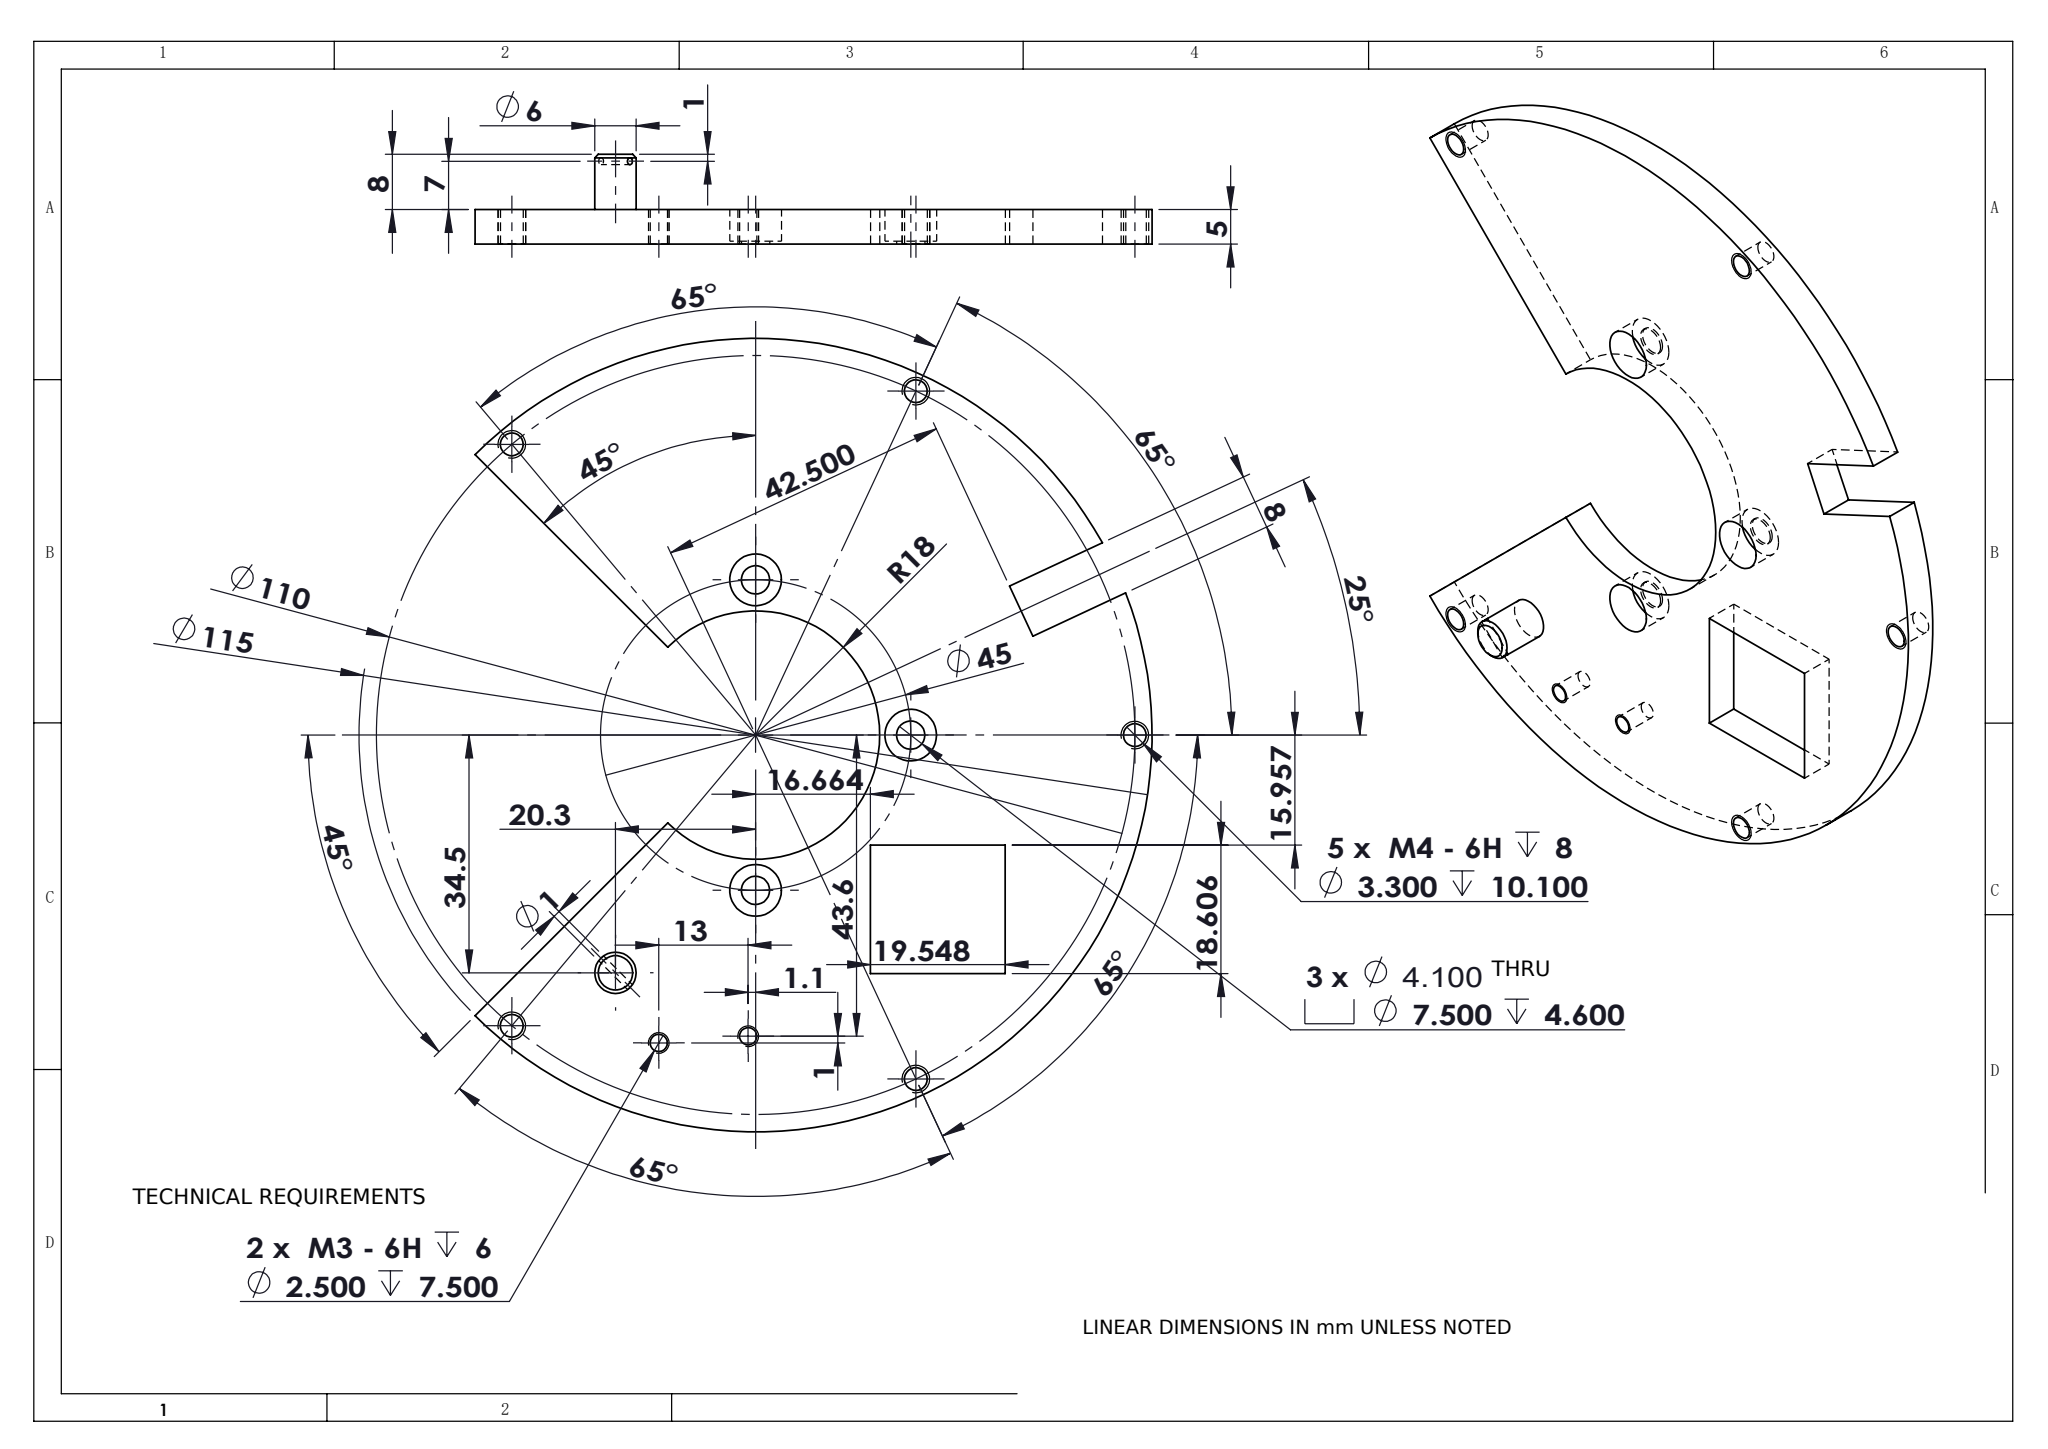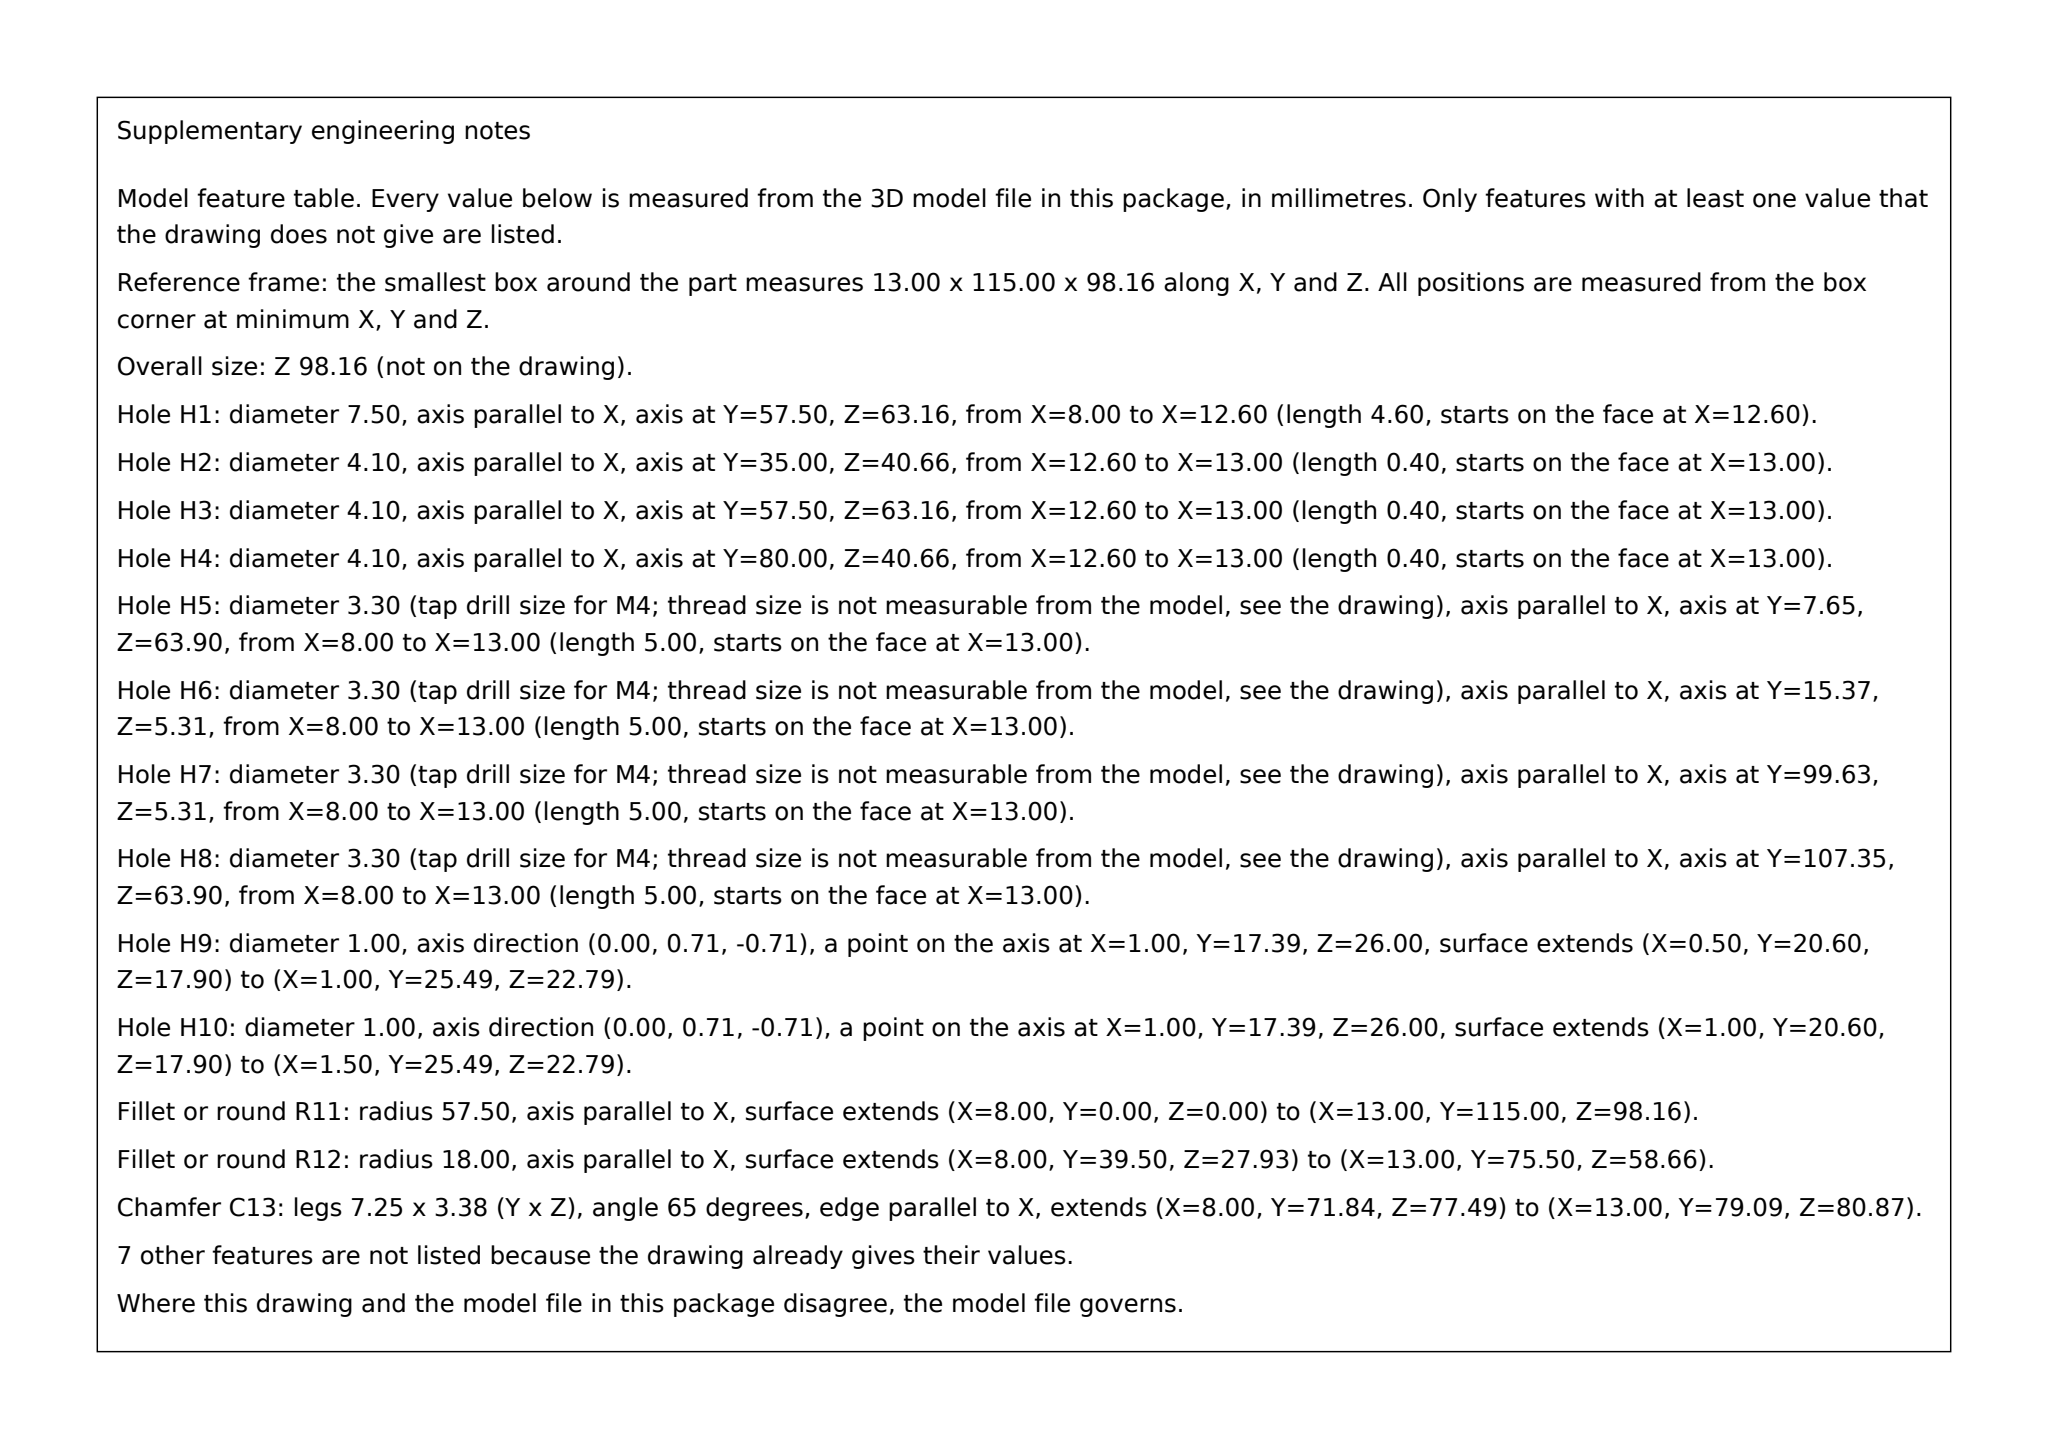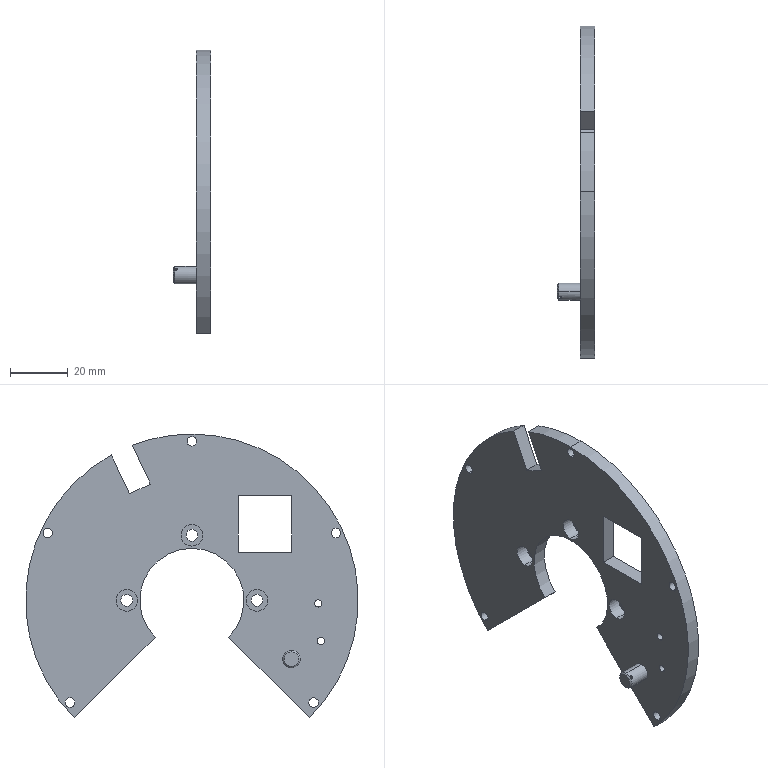Part | SolidWorks | mm | 1 solid | 52 faces | box 13 x 115 x 98.16 mm | volume 32048 mm3 | cylinder 35 | plane 15 | cone 2 | commonest cylinder face diameters 3.3 x10 7.5 x6 4.1 x6 2.5 x4 115 x3 1 x2 6 x2 36 x2